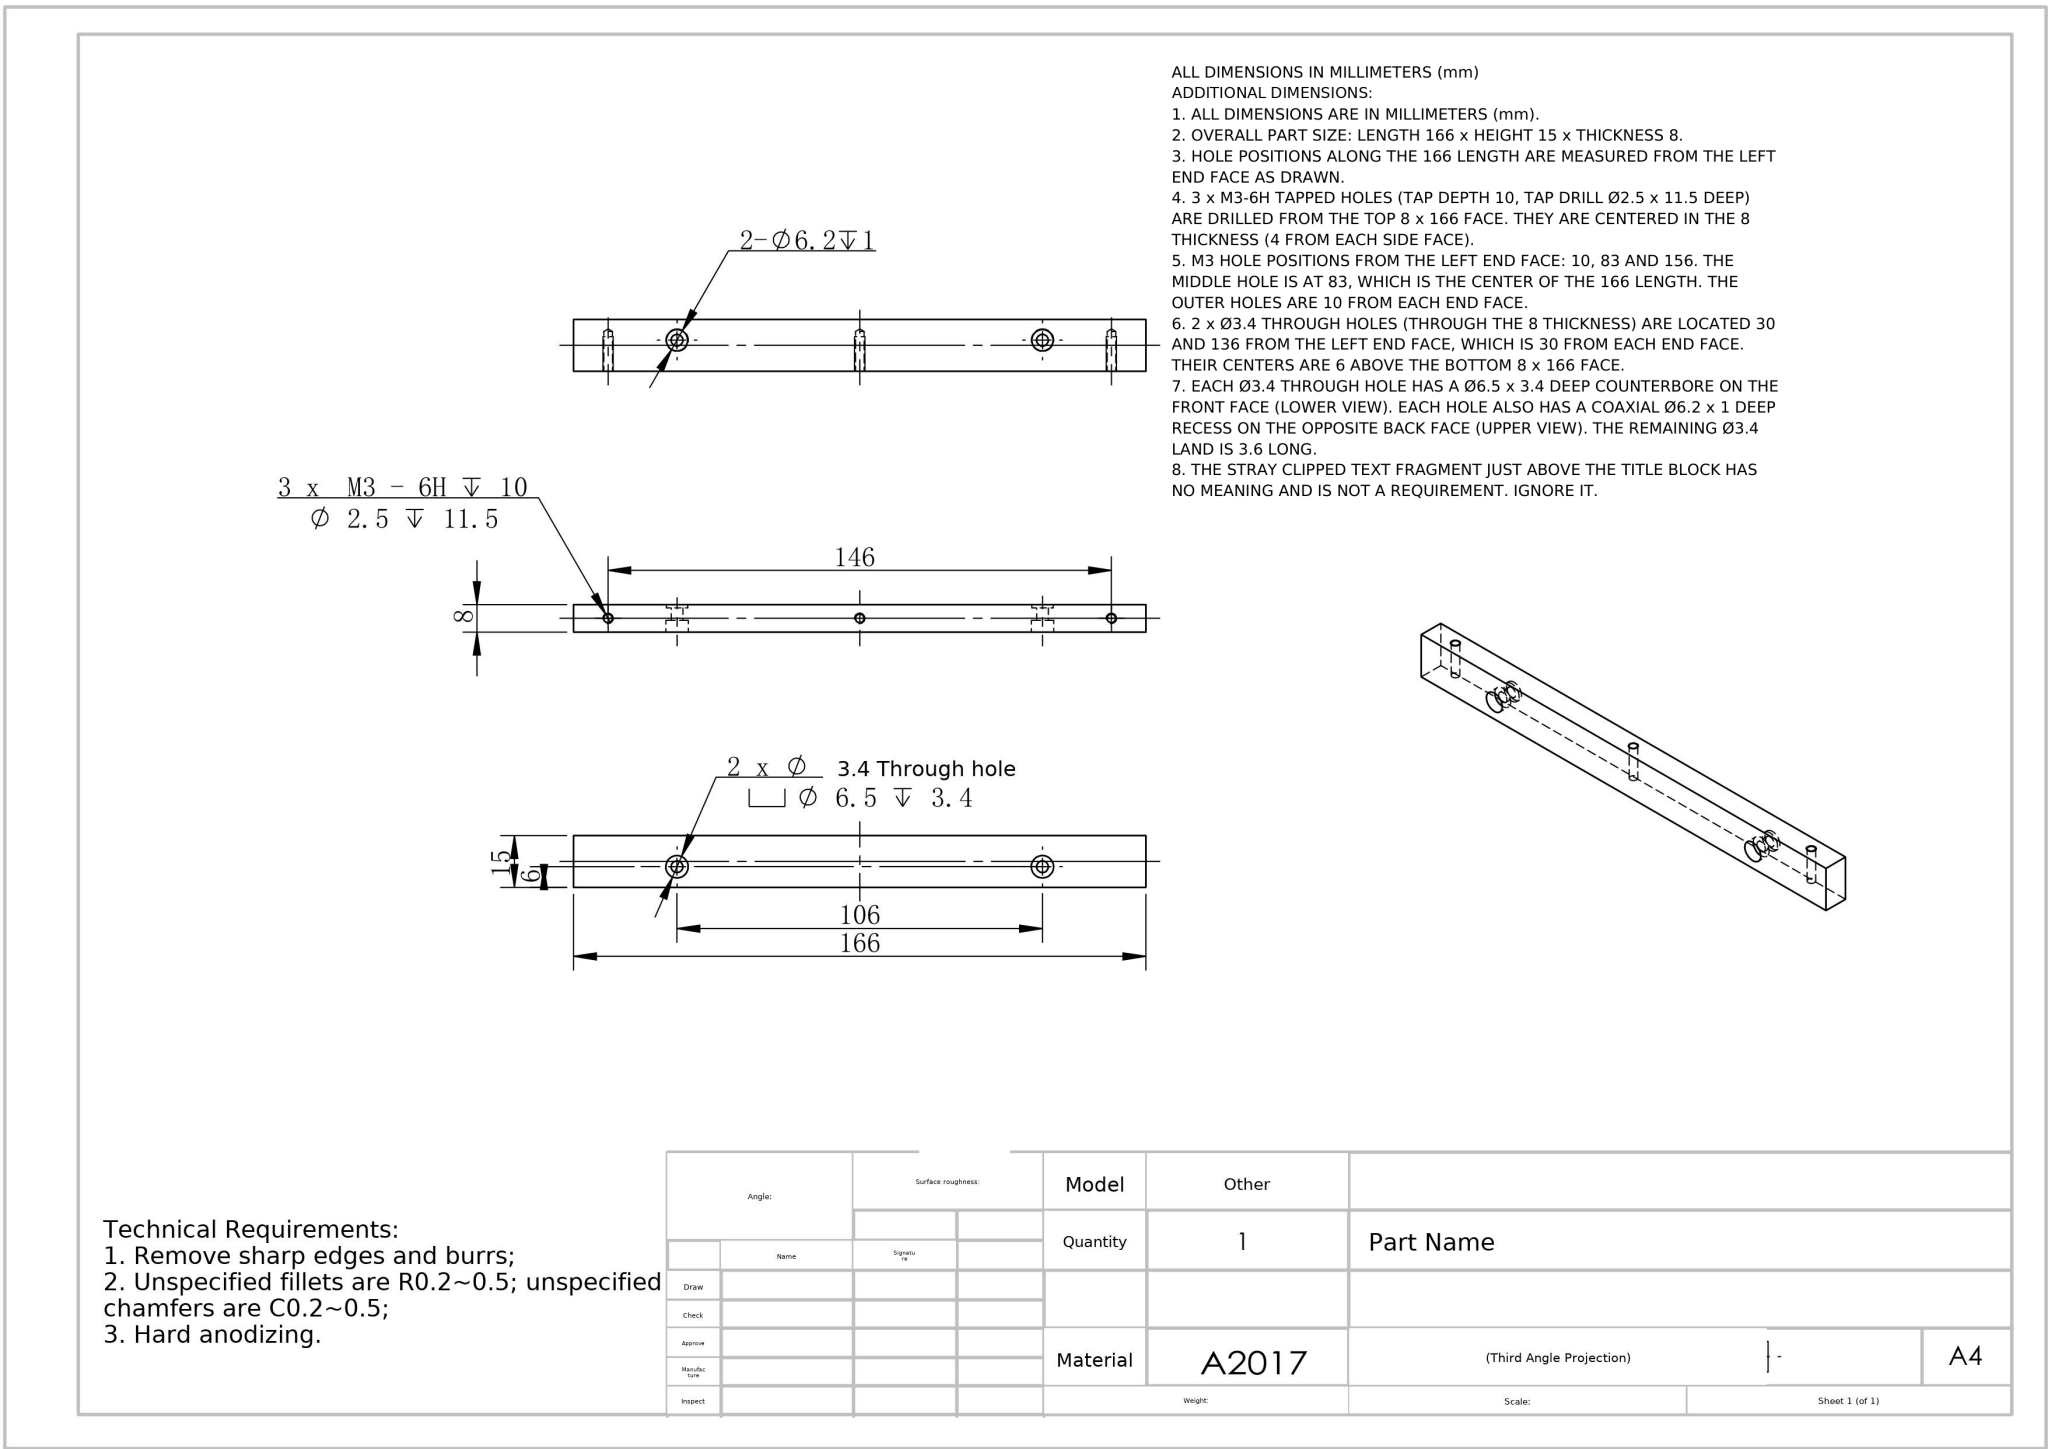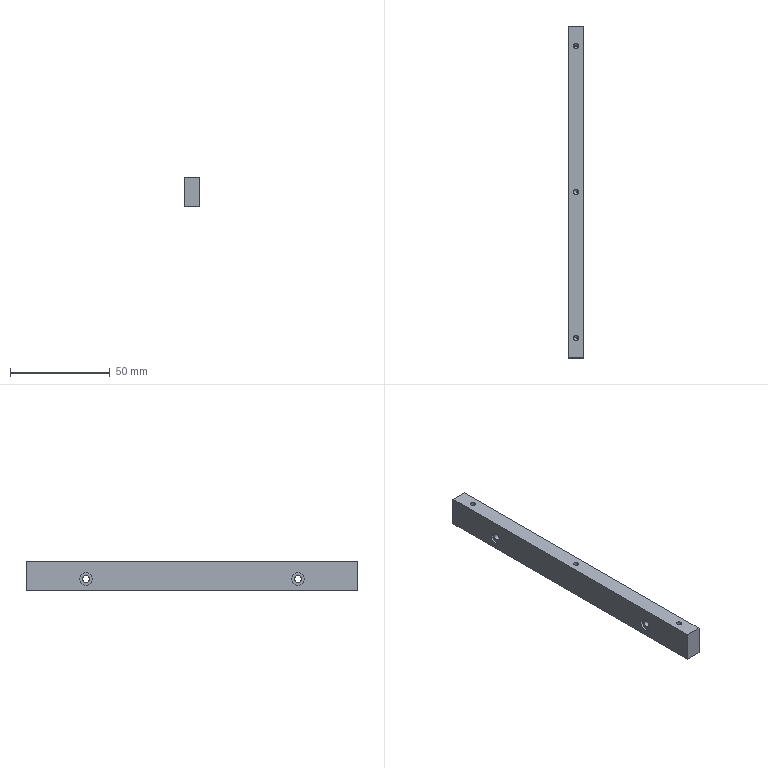Part | NX | mm | Elongated Dual-Slot Mounting Bar | 1 solid | 34 faces | box 8 x 166 x 15 mm | volume 19396 mm3 | cylinder 18 | plane 10 | cone 6 | commonest cylinder face diameters 2.5 x6 6.2 x4 6.5 x4 3.4 x4